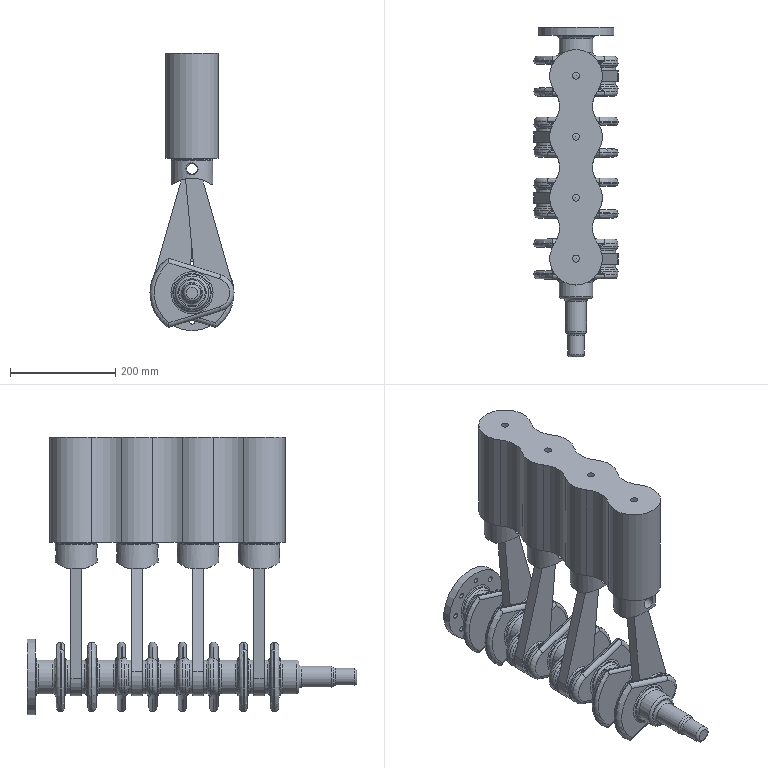Assembly | NX | mm | 10 component files | 10 solids | 397 faces | box 160 x 627 x 527.93 mm | volume 7945523 mm3 | cylinder 144 | torus 99 | plane 74 | spline 64 | cone 12 | sphere 4 | commonest cylinder face diameters 79.8 x16 16 x16 12 x16 64 x13 72 x12 100 x12 23 x8 29 x8
Bill of materials:
unnamed part 1 | 4 |  | Flat plate of constant thickness, tapered in outline, with a large round through-hole at the wide end and a small round through-hole at the narrow end; both ends are rounded around the holes.
unnamed part 2 | 1 |  | Straight extruded block whose plan outline is four overlapping circular lobes in a row, joined by concave waists. A small round hole sits at the center of each lobe.
unnamed part 3 | 1 |  | Long rotating-shaft-like part with stepped cylindrical journals along one axis and many evenly spaced flat webs set at alternating angular positions. One end has a narrow stepped shaft spigot; the other has a circular flange with a ring of small holes.
unnamed part 4 | 4 |  | Short cylindrical part with a slightly domed top, three circumferential grooves near the top, a round transverse through-bore across the body, and a lower skirt with arched cutouts on two opposite sides.
Mates:
1. touch align | multi-throw_crankshaft 1 | assembly datumplane
2. touch align | multi-throw_crankshaft 1 | assembly datumplane
3. touch align | multi-throw_crankshaft 1 | assembly datumplane
4. touch align | CONNECTING_ROD 4 face | multi-throw_crankshaft 1 face
5. center | CONNECTING_ROD 4 face | CONNECTING_ROD 4 face | multi-throw_crankshaft 1 face | multi-throw_crankshaft 1 face
6. touch align | PISTON 4 face | CONNECTING_ROD 4 face
7. center | PISTON 4 face | PISTON 4 face | CONNECTING_ROD 4 face | CONNECTING_ROD 4 face
8. touch align | CONNECTING_ROD 3 face | multi-throw_crankshaft 1 face
9. center | CONNECTING_ROD 3 face | CONNECTING_ROD 3 face | multi-throw_crankshaft 1 face | multi-throw_crankshaft 1 face
10. touch align | CONNECTING_ROD 3 face | PISTON 3 face
11. center | PISTON 3 face | PISTON 3 face | CONNECTING_ROD 3 face | CONNECTING_ROD 3 face
12. touch align | CONNECTING_ROD 2 face | multi-throw_crankshaft 1 face
13. center | CONNECTING_ROD 2 face | CONNECTING_ROD 2 face | multi-throw_crankshaft 1 face | multi-throw_crankshaft 1 face
14. touch align | PISTON 2 face | CONNECTING_ROD 2 face
15. center | PISTON 2 face | PISTON 2 face | CONNECTING_ROD 2 face | CONNECTING_ROD 2 face
16. touch align | CONNECTING_ROD 1 face | multi-throw_crankshaft 1 face
17. center | CONNECTING_ROD 1 face | CONNECTING_ROD 1 face | multi-throw_crankshaft 1 face | multi-throw_crankshaft 1 face
18. touch align | PISTON 1 face | CONNECTING_ROD 1 face
19. center | PISTON 1 face | PISTON 1 face | CONNECTING_ROD 1 face | CONNECTING_ROD 1 face
20. touch align | CYLINDER 1 datumplane | assembly datumplane
21. touch align | PISTON 4 face | CYLINDER 1 face
22. touch align | PISTON 1 face | CYLINDER 1 face
23. touch align | PISTON 2 face | CYLINDER 1 face
24. touch align | CYLINDER 1 face | PISTON 3 face
25. distance | PISTON 4 face | CYLINDER 1 face